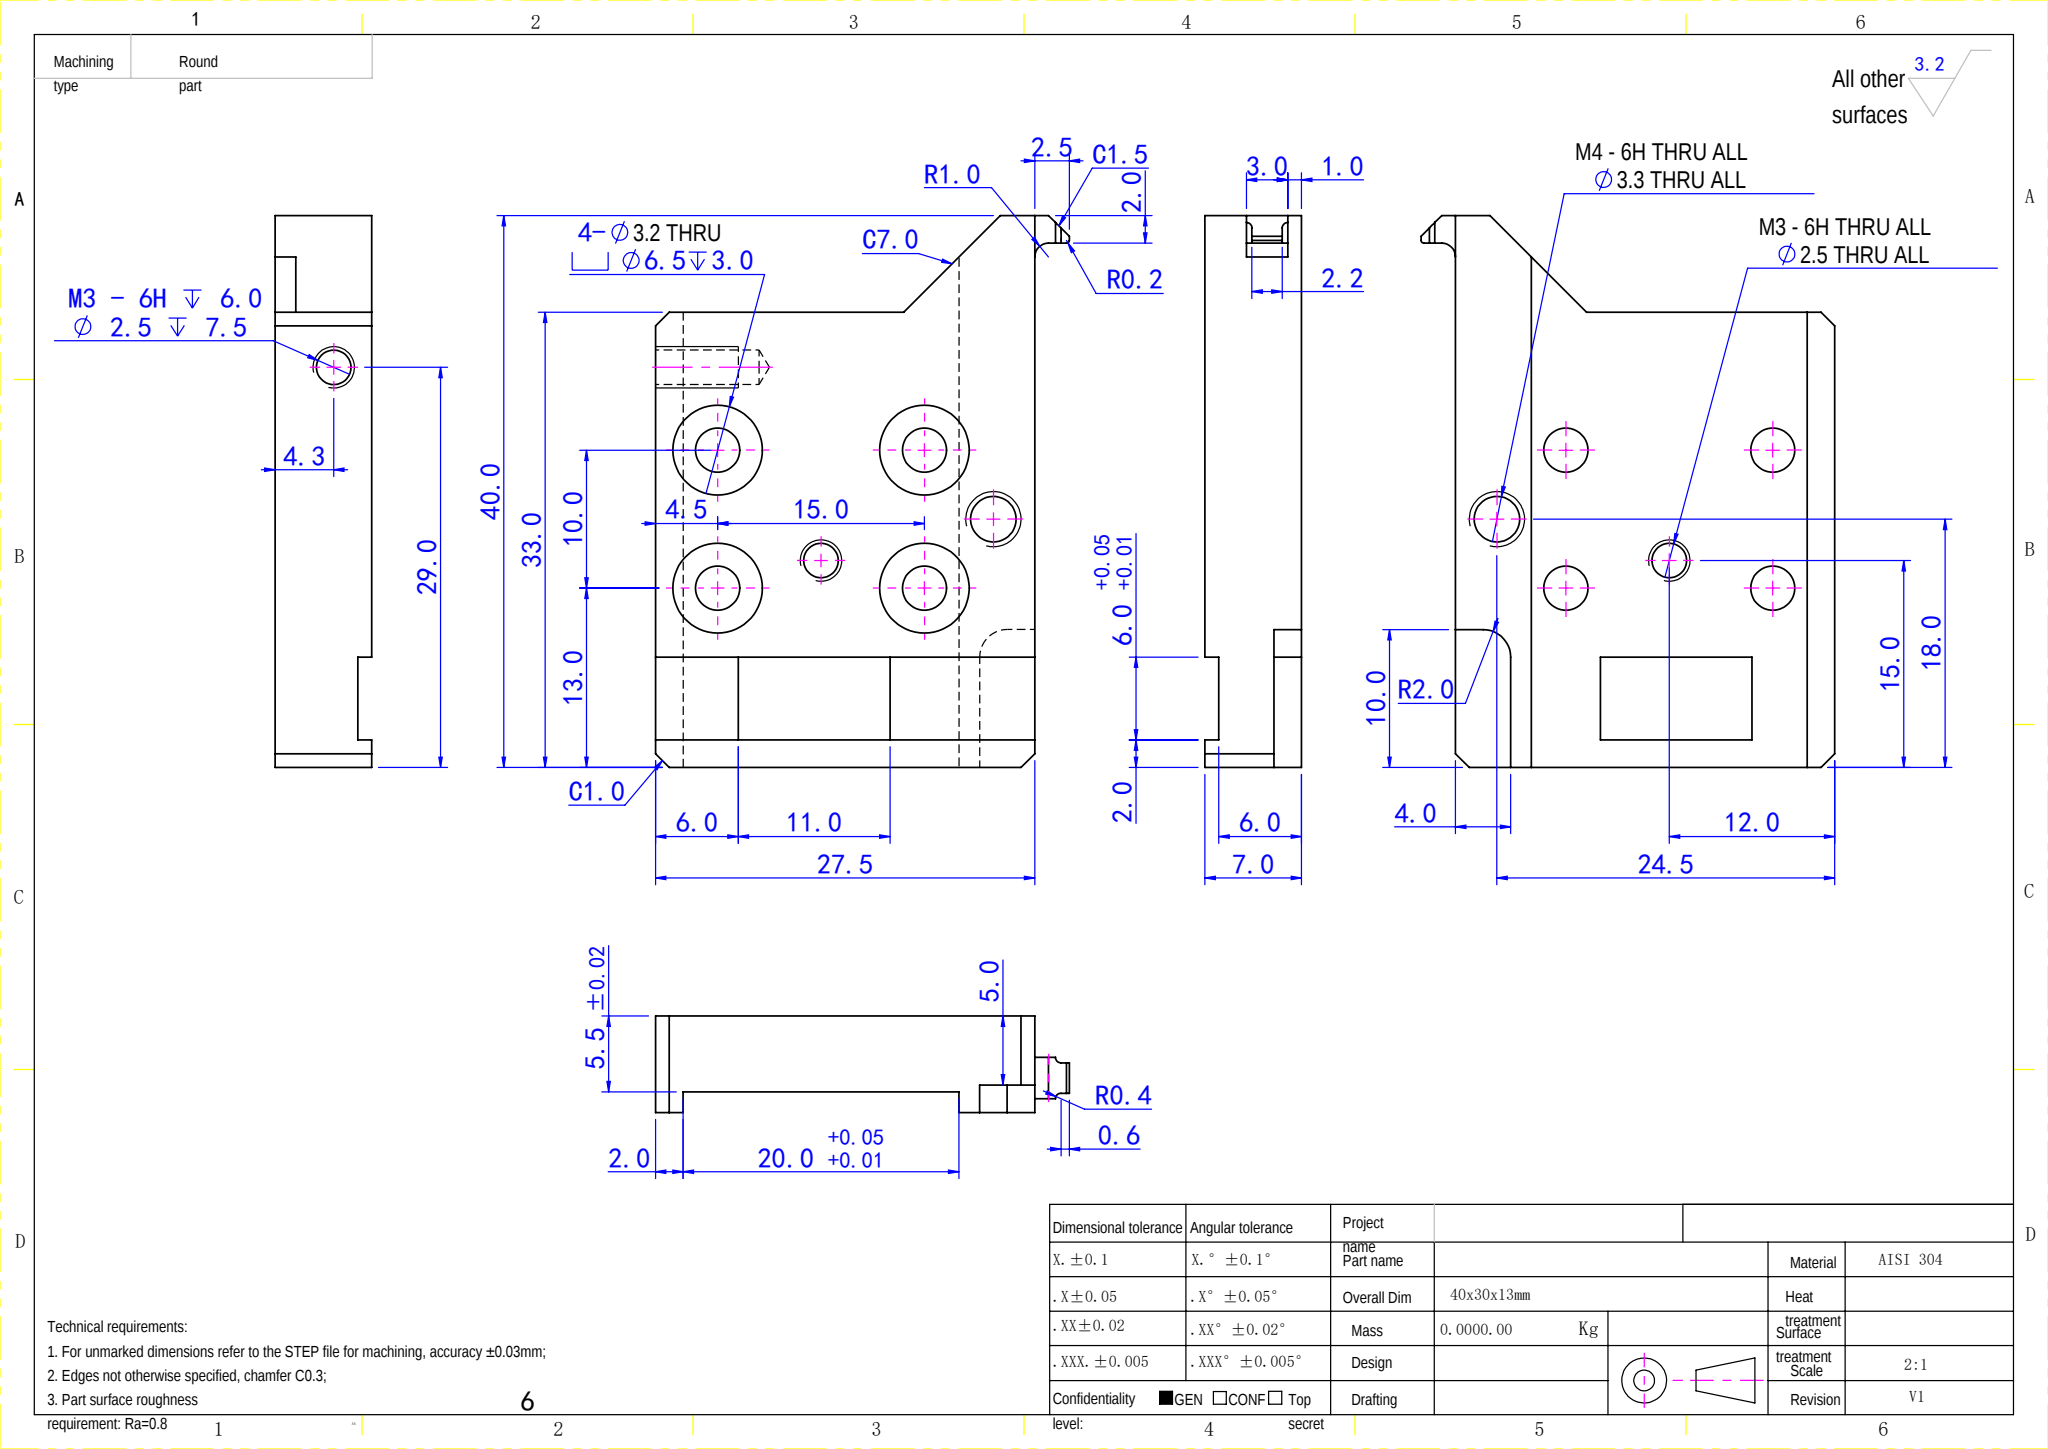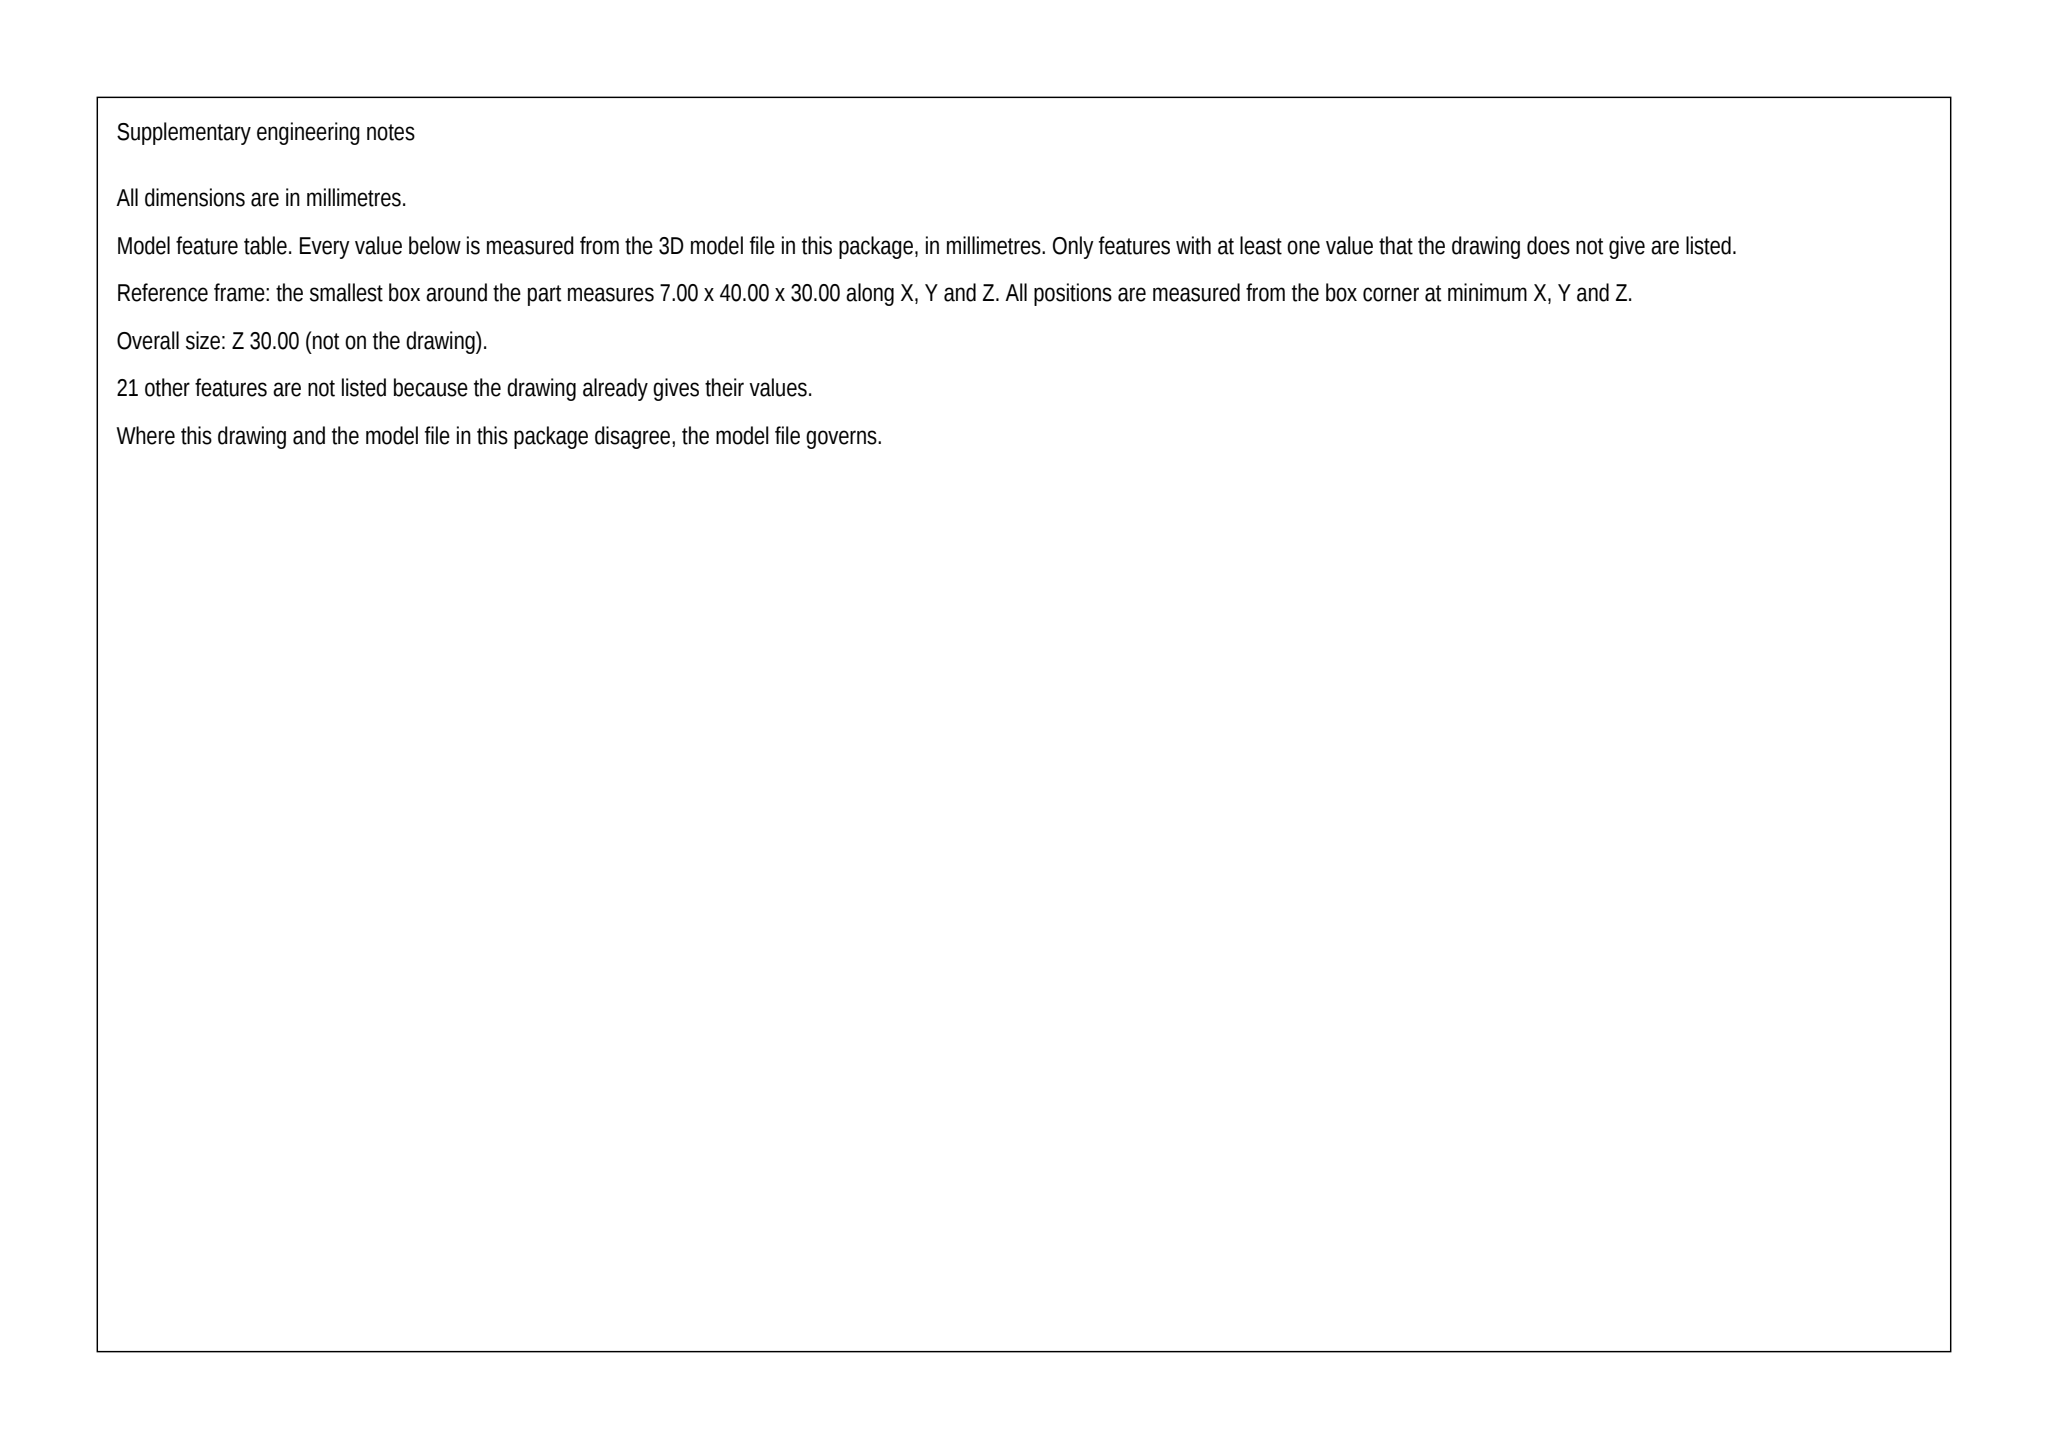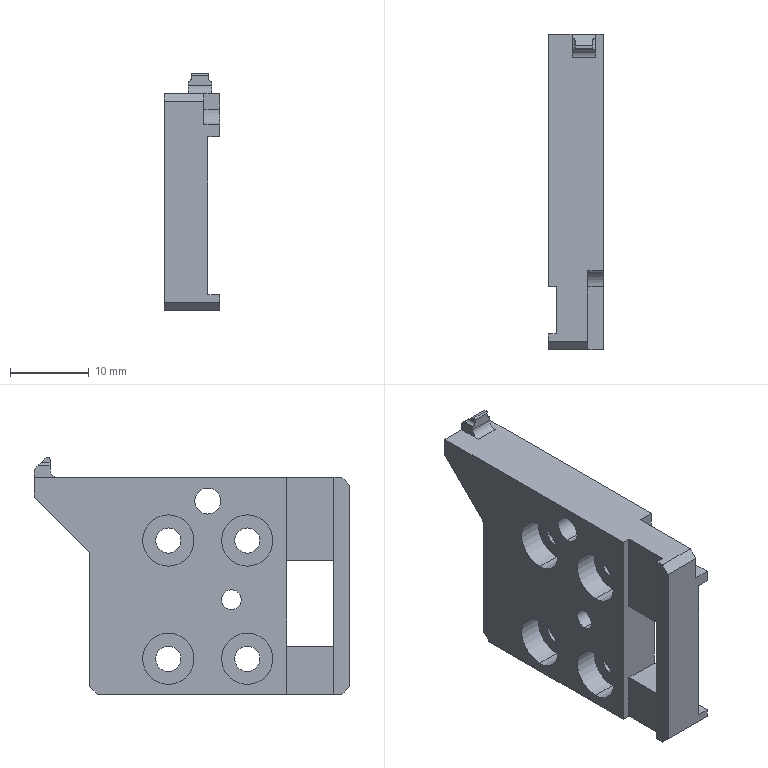Part | SolidWorks | mm | 1 solid | 65 faces | box 7 x 40 x 30 mm | volume 4503 mm3 | plane 36 | cylinder 27 | cone 2 | commonest cylinder face diameters 3.2 x8 6.5 x8 2.5 x4 3.3 x2 0.8 x2 2 x1 0.4 x1 4 x1
Drawing notes:
Ø4.0 DP 2.0 IN BACK FACE: 25.5 FROM LH EDGE, 8.0 FROM BTM | from the solid: cyl dia 4.0, axis x, pos [y=8.0, z=25.5], length 2.0
Ø2.0 DP 3.0: 28.5 FROM LH EDGE, 37.0 FROM BTM EDGE | from the solid: cyl dia 2.0, axis x, pos [y=37.0, z=28.5], length 3.0
2X Ø0.8 DP 1.5 TOP FACE, 29.4 FR LH EDGE, 3.0 & 6.0 FR FRONT | from the solid: 2 cyl dia 0.8, axis y, pos [x=3.0, z=29.4] & [x=6.0, z=29.4], len 1.5
Ø0.4 DP 2.2 CROSS HOLE: 29.8 FROM LH EDGE, 38.2 FROM BTM | from the solid: cyl dia 0.4, axis x, pos [y=38.2, z=29.8], length 2.2